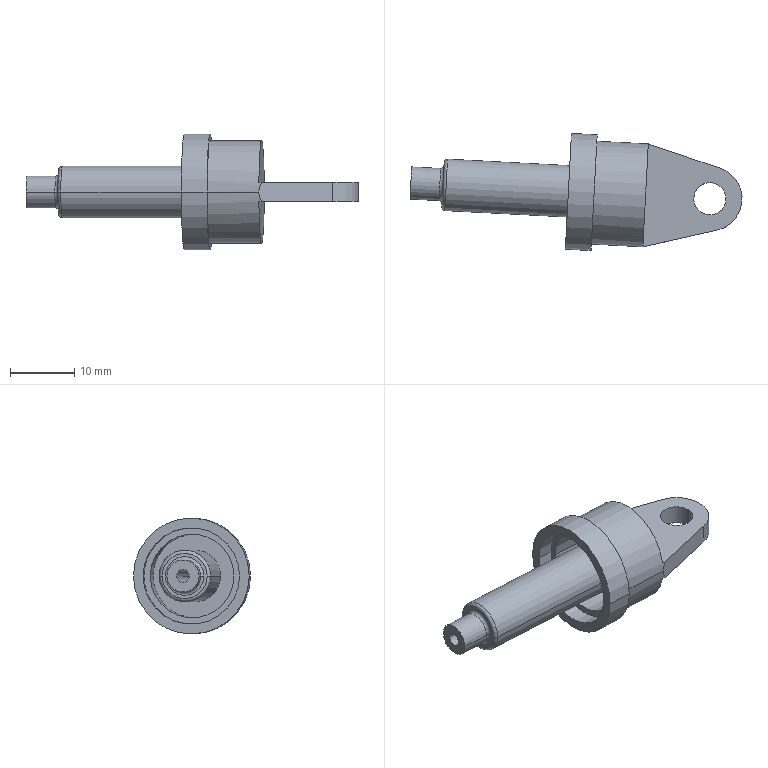Component | SolidWorks | WheelAssembly-1_DamperLowerEnd-1 | 1 solid | 34 faces | box 51.57 x 18.19 x 18 mm | volume 3074 mm3 | cylinder 17 | plane 13 | torus 4 | commonest cylinder face diameters 5 x4 2 x2 13 x2 15 x2 16 x2 18 x2 8 x2 10 x1
build123d program:
from build123d import *

# Parameters (mm, degrees)
SKETCH1_R           = 9
BOSS_EXTRUDE1_DEPTH = 12
CUT_EXTRUDE1_START  = -8
SKETCH2_R           = 9
SKETCH2_R_2         = 8
CUT_EXTRUDE1_DEPTH  = 8
SHELL1_T            = -1.5
SKETCH3_R           = 2.5
BOSS_EXTRUDE2_DEPTH = 1.5
SKETCH4_R           = 9.818
SKETCH4_R_2         = 8
CUT_EXTRUDE2_DEPTH  = 3
SKETCH5_R           = 4
SKETCH5_R_2         = 1
BOSS_EXTRUDE3_DEPTH = 35
CUT_EXTRUDE3_START  = -5
SKETCH6_R           = 4
SKETCH6_R_2         = 2.5
CUT_EXTRUDE3_DEPTH  = 5
FILLET1_R           = 0.5


with BuildPart() as part:
    # Sketch1 → Boss-Extrude1 (new body)
    with BuildSketch(Plane.XY):
        Circle(SKETCH1_R)
    extrude(amount=BOSS_EXTRUDE1_DEPTH)

    # Sketch2 → Cut-Extrude1 (cut)
    with BuildSketch(Plane.XY.offset(12).offset(CUT_EXTRUDE1_START)):
        Circle(SKETCH2_R)
        Circle(SKETCH2_R_2, mode=Mode.SUBTRACT)
    extrude(amount=CUT_EXTRUDE1_DEPTH, mode=Mode.SUBTRACT)

    # Shell1
    shell1_openings = [part.faces().sort_by_distance(p)[0] for p in [
        (0, 0, 0),
    ]]
    offset(amount=SHELL1_T, openings=shell1_openings, kind=Kind.INTERSECTION)

    # Sketch3 → Boss-Extrude2 (add, symmetric)
    with BuildSketch(Plane(origin=(0, 0, 0), x_dir=(1, 0, 0), z_dir=(0, 1, 0))):
        with BuildLine():
            Line((-8, -12), (-4.814, -23.351))
            ThreePointArc((-4.814, -23.351), (0, -27), (4.814, -23.351))
            Line((4.814, -23.351), (8, -12))
            Line((8, -12), (-8, -12))
        make_face()
        with Locations(Location((0, -22, 0), (0, 0, 270))):
            Circle(SKETCH3_R, mode=Mode.SUBTRACT)
    extrude(amount=BOSS_EXTRUDE2_DEPTH, both=True)

    # Sketch4 → Cut-Extrude2 (cut)
    with BuildSketch(Plane.XY.offset(12)):
        Circle(SKETCH4_R)
        Circle(SKETCH4_R_2, mode=Mode.SUBTRACT)
    extrude(amount=CUT_EXTRUDE2_DEPTH, mode=Mode.SUBTRACT)

    # Sketch5 → Boss-Extrude3 (add)
    with BuildSketch(Plane(origin=(0, 0, 10.5), x_dir=(-1, 0, 0), z_dir=(0, 0, -1))):
        with Locations(Location((0, 0, 0), (0, 0, 180))):
            Circle(SKETCH5_R)
        Circle(SKETCH5_R_2, mode=Mode.SUBTRACT)
    extrude(amount=BOSS_EXTRUDE3_DEPTH)

    # Sketch6 → Cut-Extrude3 (cut)
    with BuildSketch(Plane(origin=(0, 0, -24.5), x_dir=(-1, 0, 0), z_dir=(0, 0, -1)).offset(CUT_EXTRUDE3_START)):
        with Locations(Location((0, 0, 0), (0, 0, 180))):
            Circle(SKETCH6_R)
        Circle(SKETCH6_R_2, mode=Mode.SUBTRACT)
    extrude(amount=CUT_EXTRUDE3_DEPTH, mode=Mode.SUBTRACT)

    # Fillet1
    fillet1_edges = [part.edges().sort_by_distance(p)[0] for p in [
        (-4, 0, -19.5),
        (2.5, 0, -19.5),
    ]]
    fillet(fillet1_edges, radius=FILLET1_R)


solid = part.part

# Placed as in the assembly
solid = solid.moved(Location((-279.888, -132.387, -560.47), (90, 86.976, 0)))
STEP:
#1=COLOUR_RGB('',0.7922,0.8196,0.9333);
#2=FILL_AREA_STYLE_COLOUR('',#1);
#3=FILL_AREA_STYLE('',(#2));
#4=SURFACE_STYLE_FILL_AREA(#3);
#5=SURFACE_SIDE_STYLE('',(#4));
#6=SURFACE_STYLE_USAGE(.BOTH.,#5);
#7=PRESENTATION_STYLE_ASSIGNMENT((#6));
#8=CARTESIAN_POINT('',(-11.775,-5.33,-22.066));
#9=VERTEX_POINT('',#8);
#10=CARTESIAN_POINT('',(-11.758,-5.015,-22.066));
#11=VERTEX_POINT('',#10);
#12=CARTESIAN_POINT('',(-11.766,-5.173,-22.066));
#13=DIRECTION('',(0.9986,-0.05275,-0.));
#14=DIRECTION('',(0.05275,0.9986,0.));
#15=AXIS2_PLACEMENT_3D('',#12,#13,#14);
#16=CIRCLE('',#15,0.1575);
#17=EDGE_CURVE('',#9,#11,#16,.T.);
#18=ORIENTED_EDGE('',*,*,#17,.F.);
#19=CARTESIAN_POINT('',(-11.793,-5.309,-22.066));
#20=VERTEX_POINT('',#19);
#21=CARTESIAN_POINT('',(-11.773,-5.31,-22.066));
#22=DIRECTION('',(-0.,-0.,-1.));
#23=DIRECTION('',(0.,1.,0.));
#24=AXIS2_PLACEMENT_3D('',#21,#22,#23);
#25=CIRCLE('',#24,0.01969);
#26=EDGE_CURVE('',#9,#20,#25,.T.);
#27=ORIENTED_EDGE('',*,*,#26,.T.);
#28=CARTESIAN_POINT('',(-11.779,-5.034,-22.066));
#29=VERTEX_POINT('',#28);
#30=CARTESIAN_POINT('',(-11.786,-5.172,-22.066));
#31=DIRECTION('',(-0.9986,0.05275,0.));
#32=DIRECTION('',(0.05275,0.9986,0.));
#33=AXIS2_PLACEMENT_3D('',#30,#31,#32);
#34=CIRCLE('',#33,0.1378);
#35=EDGE_CURVE('',#29,#20,#34,.T.);
#36=ORIENTED_EDGE('',*,*,#35,.F.);
#37=CARTESIAN_POINT('',(-11.759,-5.035,-22.066));
#38=DIRECTION('',(0.,0.,1.));
#39=DIRECTION('',(0.,-1.,0.));
#40=AXIS2_PLACEMENT_3D('',#37,#38,#39);
#41=CIRCLE('',#40,0.01969);
#42=EDGE_CURVE('',#11,#29,#41,.T.);
#43=ORIENTED_EDGE('',*,*,#42,.F.);
#44=EDGE_LOOP('',(#18,#27,#36,#43));
#45=FACE_OUTER_BOUND('',#44,.T.);
#46=CARTESIAN_POINT('',(-11.766,-5.173,-22.066));
#47=DIRECTION('',(-0.9986,0.05275,0.));
#48=DIRECTION('',(0.05275,0.9986,-0.));
#49=AXIS2_PLACEMENT_3D('',#46,#47,#48);
#50=TOROIDAL_SURFACE('',#49,0.1378,0.01969);
#51=ADVANCED_FACE('',(#45),#50,.T.);
#52=CARTESIAN_POINT('',(-11.811,-5.269,-22.066));
#53=VERTEX_POINT('',#52);
#54=CARTESIAN_POINT('',(-11.8,-5.072,-22.066));
#55=VERTEX_POINT('',#54);
#56=CARTESIAN_POINT('',(-11.806,-5.171,-22.066));
#57=DIRECTION('',(-0.9986,0.05275,0.));
#58=DIRECTION('',(0.05275,0.9986,0.));
#59=AXIS2_PLACEMENT_3D('',#56,#57,#58);
#60=CIRCLE('',#59,0.09843);
#61=EDGE_CURVE('',#53,#55,#60,.T.);
#62=ORIENTED_EDGE('',*,*,#61,.F.);
#63=CARTESIAN_POINT('',(-11.792,-5.29,-22.066));
#64=VERTEX_POINT('',#63);
#65=CARTESIAN_POINT('',(-11.812,-5.288,-22.066));
#66=DIRECTION('',(-0.,-0.,-1.));
#67=DIRECTION('',(0.,1.,0.));
#68=AXIS2_PLACEMENT_3D('',#65,#66,#67);
#69=CIRCLE('',#68,0.01969);
#70=EDGE_CURVE('',#53,#64,#69,.T.);
#71=ORIENTED_EDGE('',*,*,#70,.T.);
#72=CARTESIAN_POINT('',(-11.78,-5.054,-22.066));
#73=VERTEX_POINT('',#72);
#74=CARTESIAN_POINT('',(-11.786,-5.172,-22.066));
#75=DIRECTION('',(0.9986,-0.05275,-0.));
#76=DIRECTION('',(0.05275,0.9986,0.));
#77=AXIS2_PLACEMENT_3D('',#74,#75,#76);
#78=CIRCLE('',#77,0.1181);
#79=EDGE_CURVE('',#73,#64,#78,.T.);
#80=ORIENTED_EDGE('',*,*,#79,.F.);
#81=CARTESIAN_POINT('',(-11.799,-5.053,-22.066));
#82=DIRECTION('',(0.,0.,1.));
#83=DIRECTION('',(0.,-1.,0.));
#84=AXIS2_PLACEMENT_3D('',#81,#82,#83);
#85=CIRCLE('',#84,0.01969);
#86=EDGE_CURVE('',#55,#73,#85,.T.);
#87=ORIENTED_EDGE('',*,*,#86,.F.);
#88=EDGE_LOOP('',(#62,#71,#80,#87));
#89=FACE_OUTER_BOUND('',#88,.T.);
#90=CARTESIAN_POINT('',(-11.806,-5.171,-22.066));
#91=DIRECTION('',(-0.9986,0.05275,0.));
#92=DIRECTION('',(0.05275,0.9986,-0.));
#93=AXIS2_PLACEMENT_3D('',#90,#91,#92);
#94=TOROIDAL_SURFACE('',#93,0.1181,0.01969);
#95=ADVANCED_FACE('',(#89),#94,.F.);
#96=CARTESIAN_POINT('',(-11.985,-5.201,-22.066));
#97=VERTEX_POINT('',#96);
#98=CARTESIAN_POINT('',(-11.98,-5.122,-22.066));
#99=VERTEX_POINT('',#98);
#100=CARTESIAN_POINT('',(-11.982,-5.161,-22.066));
#101=DIRECTION('',(-0.9986,0.05275,0.));
#102=DIRECTION('',(0.05275,0.9986,0.));
#103=AXIS2_PLACEMENT_3D('',#100,#101,#102);
#104=CIRCLE('',#103,0.03937);
#105=EDGE_CURVE('',#97,#99,#104,.T.);
#106=ORIENTED_EDGE('',*,*,#105,.T.);
#107=CARTESIAN_POINT('',(-10.604,-5.195,-22.066));
#108=VERTEX_POINT('',#107);
#109=CARTESIAN_POINT('',(-11.98,-5.122,-22.066));
#110=DIRECTION('',(0.9986,-0.05275,-0.));
#111=VECTOR('',#110,39.37);
#112=LINE('',#109,#111);
#113=EDGE_CURVE('',#99,#108,#112,.T.);
#114=ORIENTED_EDGE('',*,*,#113,.T.);
#115=CARTESIAN_POINT('',(-10.608,-5.273,-22.066));
#116=VERTEX_POINT('',#115);
#117=CARTESIAN_POINT('',(-10.606,-5.234,-22.066));
#118=DIRECTION('',(-0.9986,0.05275,0.));
#119=DIRECTION('',(0.05275,0.9986,0.));
#120=AXIS2_PLACEMENT_3D('',#117,#118,#119);
#121=CIRCLE('',#120,0.03937);
#122=EDGE_CURVE('',#116,#108,#121,.T.);
#123=ORIENTED_EDGE('',*,*,#122,.F.);
#124=CARTESIAN_POINT('',(-11.985,-5.201,-22.066));
#125=DIRECTION('',(0.9986,-0.05275,-0.));
#126=VECTOR('',#125,39.37);
#127=LINE('',#124,#126);
#128=EDGE_CURVE('',#97,#116,#127,.T.);
#129=ORIENTED_EDGE('',*,*,#128,.F.);
#130=EDGE_LOOP('',(#106,#114,#123,#129));
#131=FACE_OUTER_BOUND('',#130,.T.);
#132=CARTESIAN_POINT('',(-11.982,-5.161,-22.066));
#133=DIRECTION('',(0.9986,-0.05275,-0.));
#134=DIRECTION('',(-0.05275,-0.9986,0.));
#135=AXIS2_PLACEMENT_3D('',#132,#133,#134);
#136=CYLINDRICAL_SURFACE('',#135,0.03937);
#137=ADVANCED_FACE('',(#131),#136,.F.);
#138=CARTESIAN_POINT('',(-11.806,-5.171,-22.066));
#139=DIRECTION('',(-0.9986,0.05275,0.));
#140=DIRECTION('',(0.05275,0.9986,0.));
#141=AXIS2_PLACEMENT_3D('',#138,#139,#140);
#142=CIRCLE('',#141,0.09843);
#143=EDGE_CURVE('',#55,#53,#142,.T.);
#144=ORIENTED_EDGE('',*,*,#143,.T.);
#145=CARTESIAN_POINT('',(-11.988,-5.259,-22.066));
#146=VERTEX_POINT('',#145);
#147=CARTESIAN_POINT('',(-11.791,-5.27,-22.066));
#148=DIRECTION('',(-0.9986,0.05275,0.));
#149=VECTOR('',#148,39.37);
#150=LINE('',#147,#149);
#151=EDGE_CURVE('',#53,#146,#150,.T.);
#152=ORIENTED_EDGE('',*,*,#151,.T.);
#153=CARTESIAN_POINT('',(-11.977,-5.063,-22.066));
#154=VERTEX_POINT('',#153);
#155=CARTESIAN_POINT('',(-11.982,-5.161,-22.066));
#156=DIRECTION('',(-0.9986,0.05275,0.));
#157=DIRECTION('',(0.05275,0.9986,0.));
#158=AXIS2_PLACEMENT_3D('',#155,#156,#157);
#159=CIRCLE('',#158,0.09843);
#160=EDGE_CURVE('',#154,#146,#159,.T.);
#161=ORIENTED_EDGE('',*,*,#160,.F.);
#162=CARTESIAN_POINT('',(-11.781,-5.073,-22.066));
#163=DIRECTION('',(-0.9986,0.05275,0.));
#164=VECTOR('',#163,39.37);
#165=LINE('',#162,#164);
#166=EDGE_CURVE('',#55,#154,#165,.T.);
#167=ORIENTED_EDGE('',*,*,#166,.F.);
#168=EDGE_LOOP('',(#144,#152,#161,#167));
#169=FACE_OUTER_BOUND('',#168,.T.);
#170=CARTESIAN_POINT('',(-11.786,-5.172,-22.066));
#171=DIRECTION('',(-0.9986,0.05275,0.));
#172=DIRECTION('',(0.05275,0.9986,0.));
#173=AXIS2_PLACEMENT_3D('',#170,#171,#172);
#174=CYLINDRICAL_SURFACE('',#173,0.09843);
#175=ADVANCED_FACE('',(#169),#174,.T.);
#176=CARTESIAN_POINT('',(-10.253,-5.253,-22.125));
#177=VERTEX_POINT('',#176);
#178=CARTESIAN_POINT('',(-10.056,-5.263,-22.125));
#179=VERTEX_POINT('',#178);
#180=CARTESIAN_POINT('',(-10.154,-5.258,-22.125));
#181=DIRECTION('',(-0.,-0.,-1.));
#182=DIRECTION('',(0.9986,-0.05275,0.));
#183=AXIS2_PLACEMENT_3D('',#180,#181,#182);
#184=CIRCLE('',#183,0.09843);
#185=EDGE_CURVE('',#177,#179,#184,.T.);
#186=ORIENTED_EDGE('',*,*,#185,.T.);
#187=CARTESIAN_POINT('',(-10.056,-5.263,-22.007));
#188=VERTEX_POINT('',#187);
#189=CARTESIAN_POINT('',(-10.056,-5.263,-22.125));
#190=DIRECTION('',(0.,0.,1.));
#191=VECTOR('',#190,39.37);
#192=LINE('',#189,#191);
#193=EDGE_CURVE('',#179,#188,#192,.T.);
#194=ORIENTED_EDGE('',*,*,#193,.T.);
#195=CARTESIAN_POINT('',(-10.253,-5.253,-22.007));
#196=VERTEX_POINT('',#195);
#197=CARTESIAN_POINT('',(-10.154,-5.258,-22.007));
#198=DIRECTION('',(-0.,-0.,-1.));
#199=DIRECTION('',(0.9986,-0.05275,0.));
#200=AXIS2_PLACEMENT_3D('',#197,#198,#199);
#201=CIRCLE('',#200,0.09843);
#202=EDGE_CURVE('',#196,#188,#201,.T.);
#203=ORIENTED_EDGE('',*,*,#202,.F.);
#204=CARTESIAN_POINT('',(-10.253,-5.253,-22.125));
#205=DIRECTION('',(0.,0.,1.));
#206=VECTOR('',#205,39.37);
#207=LINE('',#204,#206);
#208=EDGE_CURVE('',#177,#196,#207,.T.);
#209=ORIENTED_EDGE('',*,*,#208,.F.);
#210=EDGE_LOOP('',(#186,#194,#203,#209));
#211=FACE_OUTER_BOUND('',#210,.T.);
#212=CARTESIAN_POINT('',(-10.154,-5.258,-22.125));
#213=DIRECTION('',(0.,0.,1.));
#214=DIRECTION('',(-0.9986,0.05275,0.));
#215=AXIS2_PLACEMENT_3D('',#212,#213,#214);
#216=CYLINDRICAL_SURFACE('',#215,0.09843);
#217=ADVANCED_FACE('',(#211),#216,.F.);
#218=CARTESIAN_POINT('',(-10.907,-4.962,-22.066));
#219=VERTEX_POINT('',#218);
#220=CARTESIAN_POINT('',(-10.934,-5.473,-22.066));
#221=VERTEX_POINT('',#220);
#222=CARTESIAN_POINT('',(-10.921,-5.217,-22.066));
#223=DIRECTION('',(0.9986,-0.05275,-0.));
#224=DIRECTION('',(-0.05275,-0.9986,0.));
#225=AXIS2_PLACEMENT_3D('',#222,#223,#224);
#226=CIRCLE('',#225,0.2559);
#227=EDGE_CURVE('',#219,#221,#226,.T.);
#228=ORIENTED_EDGE('',*,*,#227,.F.);
#229=CARTESIAN_POINT('',(-10.593,-4.978,-22.066));
#230=VERTEX_POINT('',#229);
#231=CARTESIAN_POINT('',(-10.848,-4.965,-22.066));
#232=DIRECTION('',(0.9986,-0.05275,-0.));
#233=VECTOR('',#232,39.37);
#234=LINE('',#231,#233);
#235=EDGE_CURVE('',#219,#230,#234,.T.);
#236=ORIENTED_EDGE('',*,*,#235,.T.);
#237=CARTESIAN_POINT('',(-10.62,-5.489,-22.066));
#238=VERTEX_POINT('',#237);
#239=CARTESIAN_POINT('',(-10.606,-5.234,-22.066));
#240=DIRECTION('',(0.9986,-0.05275,-0.));
#241=DIRECTION('',(-0.05275,-0.9986,0.));
#242=AXIS2_PLACEMENT_3D('',#239,#240,#241);
#243=CIRCLE('',#242,0.2559);
#244=EDGE_CURVE('',#230,#238,#243,.T.);
#245=ORIENTED_EDGE('',*,*,#244,.T.);
#246=CARTESIAN_POINT('',(-10.875,-5.476,-22.066));
#247=DIRECTION('',(0.9986,-0.05275,-0.));
#248=VECTOR('',#247,39.37);
#249=LINE('',#246,#248);
#250=EDGE_CURVE('',#221,#238,#249,.T.);
#251=ORIENTED_EDGE('',*,*,#250,.F.);
#252=EDGE_LOOP('',(#228,#236,#245,#251));
#253=FACE_OUTER_BOUND('',#252,.T.);
#254=CARTESIAN_POINT('',(-10.862,-5.22,-22.066));
#255=DIRECTION('',(0.9986,-0.05275,-0.));
#256=DIRECTION('',(-0.05275,-0.9986,0.));
#257=AXIS2_PLACEMENT_3D('',#254,#255,#256);
#258=CYLINDRICAL_SURFACE('',#257,0.2559);
#259=ADVANCED_FACE('',(#253),#258,.F.);
#260=CARTESIAN_POINT('',(-10.905,-4.922,-22.066));
#261=VERTEX_POINT('',#260);
#262=CARTESIAN_POINT('',(-10.937,-5.512,-22.066));
#263=VERTEX_POINT('',#262);
#264=CARTESIAN_POINT('',(-10.921,-5.217,-22.066));
#265=DIRECTION('',(0.9986,-0.05275,-0.));
#266=DIRECTION('',(-0.05275,-0.9986,0.));
#267=AXIS2_PLACEMENT_3D('',#264,#265,#266);
#268=CIRCLE('',#267,0.2953);
#269=EDGE_CURVE('',#261,#263,#268,.T.);
#270=ORIENTED_EDGE('',*,*,#269,.T.);
#271=CARTESIAN_POINT('',(-11.035,-5.507,-22.066));
#272=VERTEX_POINT('',#271);
#273=CARTESIAN_POINT('',(-10.563,-5.532,-22.066));
#274=DIRECTION('',(-0.9986,0.05275,0.));
#275=VECTOR('',#274,39.37);
#276=LINE('',#273,#275);
#277=EDGE_CURVE('',#263,#272,#276,.T.);
#278=ORIENTED_EDGE('',*,*,#277,.T.);
#279=CARTESIAN_POINT('',(-11.004,-4.917,-22.066));
#280=VERTEX_POINT('',#279);
#281=CARTESIAN_POINT('',(-11.019,-5.212,-22.066));
#282=DIRECTION('',(0.9986,-0.05275,-0.));
#283=DIRECTION('',(-0.05275,-0.9986,0.));
#284=AXIS2_PLACEMENT_3D('',#281,#282,#283);
#285=CIRCLE('',#284,0.2953);
#286=EDGE_CURVE('',#280,#272,#285,.T.);
#287=ORIENTED_EDGE('',*,*,#286,.F.);
#288=CARTESIAN_POINT('',(-10.532,-4.942,-22.066));
#289=DIRECTION('',(-0.9986,0.05275,0.));
#290=VECTOR('',#289,39.37);
#291=LINE('',#288,#290);
#292=EDGE_CURVE('',#261,#280,#291,.T.);
#293=ORIENTED_EDGE('',*,*,#292,.F.);
#294=EDGE_LOOP('',(#270,#278,#287,#293));
#295=FACE_OUTER_BOUND('',#294,.T.);
#296=CARTESIAN_POINT('',(-10.547,-5.237,-22.066));
#297=DIRECTION('',(-0.9986,0.05275,0.));
#298=DIRECTION('',(0.05275,0.9986,0.));
#299=AXIS2_PLACEMENT_3D('',#296,#297,#298);
#300=CYLINDRICAL_SURFACE('',#299,0.2953);
#301=ADVANCED_FACE('',(#295),#300,.F.);
#302=CARTESIAN_POINT('',(-10.879,-5.535,-22.066));
#303=VERTEX_POINT('',#302);
#304=CARTESIAN_POINT('',(-10.845,-4.906,-22.066));
#305=VERTEX_POINT('',#304);
#306=CARTESIAN_POINT('',(-10.862,-5.22,-22.066));
#307=DIRECTION('',(0.9986,-0.05275,-0.));
#308=DIRECTION('',(-0.05275,-0.9986,0.));
#309=AXIS2_PLACEMENT_3D('',#306,#307,#308);
#310=CIRCLE('',#309,0.315);
#311=EDGE_CURVE('',#303,#305,#310,.T.);
#312=ORIENTED_EDGE('',*,*,#311,.T.);
#313=CARTESIAN_POINT('',(-10.531,-4.922,-22.066));
#314=VERTEX_POINT('',#313);
#315=CARTESIAN_POINT('',(-10.845,-4.906,-22.066));
#316=DIRECTION('',(0.9986,-0.05275,-0.));
#317=VECTOR('',#316,39.37);
#318=LINE('',#315,#317);
#319=EDGE_CURVE('',#305,#314,#318,.T.);
#320=ORIENTED_EDGE('',*,*,#319,.T.);
#321=CARTESIAN_POINT('',(-10.511,-4.929,-22.125));
#322=VERTEX_POINT('',#321);
#323=CARTESIAN_POINT('',(-10.511,-4.929,-22.125));
#324=CARTESIAN_POINT('',(-10.524,-4.925,-22.105));
#325=CARTESIAN_POINT('',(-10.531,-4.922,-22.086));
#326=CARTESIAN_POINT('',(-10.531,-4.922,-22.066));
#327=(BOUNDED_CURVE()B_SPLINE_CURVE(3,(#323,#324,#325,#326),.UNSPECIFIED.,.F.,.F.)B_SPLINE_CURVE_WITH_KNOTS((4,4),(6.095,6.283),.UNSPECIFIED.)CURVE()GEOMETRIC_REPRESENTATION_ITEM()RATIONAL_B_SPLINE_CURVE((1.,0.997,0.997,1.))REPRESENTATION_ITEM(''));
#328=EDGE_CURVE('',#322,#314,#327,.T.);
#329=ORIENTED_EDGE('',*,*,#328,.F.);
#330=CARTESIAN_POINT('',(-10.531,-4.928,-22.125));
#331=VERTEX_POINT('',#330);
#332=CARTESIAN_POINT('',(-10.413,-4.934,-22.125));
#333=DIRECTION('',(-0.9986,0.05275,0.));
#334=VECTOR('',#333,39.37);
#335=LINE('',#332,#334);
#336=EDGE_CURVE('',#322,#331,#335,.T.);
#337=ORIENTED_EDGE('',*,*,#336,.T.);
#338=CARTESIAN_POINT('',(-10.564,-5.546,-22.125));
#339=VERTEX_POINT('',#338);
#340=CARTESIAN_POINT('',(-10.547,-5.237,-22.066));
#341=DIRECTION('',(0.9986,-0.05275,-0.));
#342=DIRECTION('',(-0.05275,-0.9986,0.));
#343=AXIS2_PLACEMENT_3D('',#340,#341,#342);
#344=CIRCLE('',#343,0.315);
#345=EDGE_CURVE('',#339,#331,#344,.T.);
#346=ORIENTED_EDGE('',*,*,#345,.F.);
#347=CARTESIAN_POINT('',(-10.544,-5.547,-22.125));
#348=VERTEX_POINT('',#347);
#349=CARTESIAN_POINT('',(-10.446,-5.552,-22.125));
#350=DIRECTION('',(0.9986,-0.05275,-0.));
#351=VECTOR('',#350,39.37);
#352=LINE('',#349,#351);
#353=EDGE_CURVE('',#339,#348,#352,.T.);
#354=ORIENTED_EDGE('',*,*,#353,.T.);
#355=CARTESIAN_POINT('',(-10.564,-5.552,-22.066));
#356=VERTEX_POINT('',#355);
#357=CARTESIAN_POINT('',(-10.564,-5.552,-22.066));
#358=CARTESIAN_POINT('',(-10.564,-5.552,-22.086));
#359=CARTESIAN_POINT('',(-10.557,-5.55,-22.105));
#360=CARTESIAN_POINT('',(-10.544,-5.547,-22.125));
#361=(BOUNDED_CURVE()B_SPLINE_CURVE(3,(#357,#358,#359,#360),.UNSPECIFIED.,.F.,.F.)B_SPLINE_CURVE_WITH_KNOTS((4,4),(0.,0.1886),.UNSPECIFIED.)CURVE()GEOMETRIC_REPRESENTATION_ITEM()RATIONAL_B_SPLINE_CURVE((1.,0.997,0.997,1.))REPRESENTATION_ITEM(''));
#362=EDGE_CURVE('',#356,#348,#361,.T.);
#363=ORIENTED_EDGE('',*,*,#362,.F.);
#364=CARTESIAN_POINT('',(-10.879,-5.535,-22.066));
#365=DIRECTION('',(0.9986,-0.05275,-0.));
#366=VECTOR('',#365,39.37);
#367=LINE('',#364,#366);
#368=EDGE_CURVE('',#303,#356,#367,.T.);
#369=ORIENTED_EDGE('',*,*,#368,.F.);
#370=EDGE_LOOP('',(#312,#320,#329,#337,#346,#354,#363,#369));
#371=FACE_OUTER_BOUND('',#370,.T.);
#372=CARTESIAN_POINT('',(-10.862,-5.22,-22.066));
#373=DIRECTION('',(0.9986,-0.05275,-0.));
#374=DIRECTION('',(-0.05275,-0.9986,0.));
#375=AXIS2_PLACEMENT_3D('',#372,#373,#374);
#376=CYLINDRICAL_SURFACE('',#375,0.315);
#377=ADVANCED_FACE('',(#371),#376,.T.);
#378=CARTESIAN_POINT('',(-10.881,-5.574,-22.066));
#379=VERTEX_POINT('',#378);
#380=CARTESIAN_POINT('',(-10.843,-4.867,-22.066));
#381=VERTEX_POINT('',#380);
#382=CARTESIAN_POINT('',(-10.862,-5.22,-22.066));
#383=DIRECTION('',(0.9986,-0.05275,-0.));
#384=DIRECTION('',(-0.05275,-0.9986,0.));
#385=AXIS2_PLACEMENT_3D('',#382,#383,#384);
#386=CIRCLE('',#385,0.3543);
#387=EDGE_CURVE('',#379,#381,#386,.T.);
#388=ORIENTED_EDGE('',*,*,#387,.F.);
#389=CARTESIAN_POINT('',(-11.038,-5.566,-22.066));
#390=VERTEX_POINT('',#389);
#391=CARTESIAN_POINT('',(-10.566,-5.591,-22.066));
#392=DIRECTION('',(-0.9986,0.05275,0.));
#393=VECTOR('',#392,39.37);
#394=LINE('',#391,#393);
#395=EDGE_CURVE('',#379,#390,#394,.T.);
#396=ORIENTED_EDGE('',*,*,#395,.T.);
#397=CARTESIAN_POINT('',(-11.001,-4.858,-22.066));
#398=VERTEX_POINT('',#397);
#399=CARTESIAN_POINT('',(-11.019,-5.212,-22.066));
#400=DIRECTION('',(0.9986,-0.05275,-0.));
#401=DIRECTION('',(-0.05275,-0.9986,0.));
#402=AXIS2_PLACEMENT_3D('',#399,#400,#401);
#403=CIRCLE('',#402,0.3543);
#404=EDGE_CURVE('',#390,#398,#403,.T.);
#405=ORIENTED_EDGE('',*,*,#404,.T.);
#406=CARTESIAN_POINT('',(-10.529,-4.883,-22.066));
#407=DIRECTION('',(-0.9986,0.05275,0.));
#408=VECTOR('',#407,39.37);
#409=LINE('',#406,#408);
#410=EDGE_CURVE('',#381,#398,#409,.T.);
#411=ORIENTED_EDGE('',*,*,#410,.F.);
#412=EDGE_LOOP('',(#388,#396,#405,#411));
#413=FACE_OUTER_BOUND('',#412,.T.);
#414=CARTESIAN_POINT('',(-10.547,-5.237,-22.066));
#415=DIRECTION('',(-0.9986,0.05275,0.));
#416=DIRECTION('',(0.05275,0.9986,0.));
#417=AXIS2_PLACEMENT_3D('',#414,#415,#416);
#418=CYLINDRICAL_SURFACE('',#417,0.3543);
#419=ADVANCED_FACE('',(#413),#418,.T.);
#420=ORIENTED_EDGE('',*,*,#17,.T.);
#421=CARTESIAN_POINT('',(-10.598,-5.077,-22.066));
#422=VERTEX_POINT('',#421);
#423=CARTESIAN_POINT('',(-11.974,-5.004,-22.066));
#424=DIRECTION('',(0.9986,-0.05275,-0.));
#425=VECTOR('',#424,39.37);
#426=LINE('',#423,#425);
#427=EDGE_CURVE('',#11,#422,#426,.T.);
#428=ORIENTED_EDGE('',*,*,#427,.T.);
#429=CARTESIAN_POINT('',(-10.615,-5.391,-22.066));
#430=VERTEX_POINT('',#429);
#431=CARTESIAN_POINT('',(-10.606,-5.234,-22.066));
#432=DIRECTION('',(-0.9986,0.05275,0.));
#433=DIRECTION('',(-0.05275,-0.9986,0.));
#434=AXIS2_PLACEMENT_3D('',#431,#432,#433);
#435=CIRCLE('',#434,0.1575);
#436=EDGE_CURVE('',#422,#430,#435,.T.);
#437=ORIENTED_EDGE('',*,*,#436,.T.);
#438=CARTESIAN_POINT('',(-11.991,-5.318,-22.066));
#439=DIRECTION('',(0.9986,-0.05275,-0.));
#440=VECTOR('',#439,39.37);
#441=LINE('',#438,#440);
#442=EDGE_CURVE('',#9,#430,#441,.T.);
#443=ORIENTED_EDGE('',*,*,#442,.F.);
#444=EDGE_LOOP('',(#420,#428,#437,#443));
#445=FACE_OUTER_BOUND('',#444,.T.);
#446=CARTESIAN_POINT('',(-11.982,-5.161,-22.066));
#447=DIRECTION('',(0.9986,-0.05275,-0.));
#448=DIRECTION('',(-0.05275,-0.9986,0.));
#449=AXIS2_PLACEMENT_3D('',#446,#447,#448);
#450=CYLINDRICAL_SURFACE('',#449,0.1575);
#451=ADVANCED_FACE('',(#445),#450,.T.);
#452=ORIENTED_EDGE('',*,*,#427,.F.);
#453=CARTESIAN_POINT('',(-11.766,-5.173,-22.066));
#454=DIRECTION('',(0.9986,-0.05275,-0.));
#455=DIRECTION('',(0.05275,0.9986,0.));
#456=AXIS2_PLACEMENT_3D('',#453,#454,#455);
#457=CIRCLE('',#456,0.1575);
#458=EDGE_CURVE('',#11,#9,#457,.T.);
#459=ORIENTED_EDGE('',*,*,#458,.T.);
#460=ORIENTED_EDGE('',*,*,#442,.T.);
#461=CARTESIAN_POINT('',(-10.606,-5.234,-22.066));
#462=DIRECTION('',(-0.9986,0.05275,0.));
#463=DIRECTION('',(-0.05275,-0.9986,0.));
#464=AXIS2_PLACEMENT_3D('',#461,#462,#463);
#465=CIRCLE('',#464,0.1575);
#466=EDGE_CURVE('',#430,#422,#465,.T.);
#467=ORIENTED_EDGE('',*,*,#466,.T.);
#468=EDGE_LOOP('',(#452,#459,#460,#467));
#469=FACE_OUTER_BOUND('',#468,.T.);
#470=CARTESIAN_POINT('',(-11.982,-5.161,-22.066));
#471=DIRECTION('',(0.9986,-0.05275,-0.));
#472=DIRECTION('',(-0.05275,-0.9986,0.));
#473=AXIS2_PLACEMENT_3D('',#470,#471,#472);
#474=CYLINDRICAL_SURFACE('',#473,0.1575);
#475=ADVANCED_FACE('',(#469),#474,.T.);
#476=CARTESIAN_POINT('',(-10.091,-5.071,-22.125));
#477=VERTEX_POINT('',#476);
#478=CARTESIAN_POINT('',(-10.531,-4.922,-22.125));
#479=DIRECTION('',(0.9472,-0.3206,0.));
#480=VECTOR('',#479,39.37);
#481=LINE('',#478,#480);
#482=EDGE_CURVE('',#322,#477,#481,.T.);
#483=ORIENTED_EDGE('',*,*,#482,.F.);
#484=ORIENTED_EDGE('',*,*,#328,.T.);
#485=CARTESIAN_POINT('',(-10.511,-4.929,-22.007));
#486=VERTEX_POINT('',#485);
#487=CARTESIAN_POINT('',(-10.531,-4.922,-22.066));
#488=CARTESIAN_POINT('',(-10.531,-4.922,-22.046));
#489=CARTESIAN_POINT('',(-10.524,-4.925,-22.026));
#490=CARTESIAN_POINT('',(-10.511,-4.929,-22.007));
#491=(BOUNDED_CURVE()B_SPLINE_CURVE(3,(#487,#488,#489,#490),.UNSPECIFIED.,.F.,.F.)B_SPLINE_CURVE_WITH_KNOTS((4,4),(0.,0.1886),.UNSPECIFIED.)CURVE()GEOMETRIC_REPRESENTATION_ITEM()RATIONAL_B_SPLINE_CURVE((1.,0.997,0.997,1.))REPRESENTATION_ITEM(''));
#492=EDGE_CURVE('',#314,#486,#491,.T.);
#493=ORIENTED_EDGE('',*,*,#492,.T.);
#494=CARTESIAN_POINT('',(-10.091,-5.071,-22.007));
#495=VERTEX_POINT('',#494);
#496=CARTESIAN_POINT('',(-10.531,-4.922,-22.007));
#497=DIRECTION('',(0.9472,-0.3206,0.));
#498=VECTOR('',#497,39.37);
#499=LINE('',#496,#498);
#500=EDGE_CURVE('',#486,#495,#499,.T.);
#501=ORIENTED_EDGE('',*,*,#500,.T.);
#502=CARTESIAN_POINT('',(-10.091,-5.071,-22.125));
#503=DIRECTION('',(0.,0.,1.));
#504=VECTOR('',#503,39.37);
#505=LINE('',#502,#504);
#506=EDGE_CURVE('',#477,#495,#505,.T.);
#507=ORIENTED_EDGE('',*,*,#506,.F.);
#508=EDGE_LOOP('',(#483,#484,#493,#501,#507));
#509=FACE_OUTER_BOUND('',#508,.T.);
#510=CARTESIAN_POINT('',(-10.531,-4.922,-22.125));
#511=DIRECTION('',(-0.3206,-0.9472,0.));
#512=DIRECTION('',(-0.9472,0.3206,-0.));
#513=AXIS2_PLACEMENT_3D('',#510,#511,#512);
#514=PLANE('',#513);
#515=ADVANCED_FACE('',(#509),#514,.F.);
#516=CARTESIAN_POINT('',(-10.544,-5.547,-22.007));
#517=VERTEX_POINT('',#516);
#518=CARTESIAN_POINT('',(-10.544,-5.547,-22.007));
#519=CARTESIAN_POINT('',(-10.557,-5.55,-22.026));
#520=CARTESIAN_POINT('',(-10.564,-5.552,-22.046));
#521=CARTESIAN_POINT('',(-10.564,-5.552,-22.066));
#522=(BOUNDED_CURVE()B_SPLINE_CURVE(3,(#518,#519,#520,#521),.UNSPECIFIED.,.F.,.F.)B_SPLINE_CURVE_WITH_KNOTS((4,4),(6.095,6.283),.UNSPECIFIED.)CURVE()GEOMETRIC_REPRESENTATION_ITEM()RATIONAL_B_SPLINE_CURVE((1.,0.997,0.997,1.))REPRESENTATION_ITEM(''));
#523=EDGE_CURVE('',#517,#356,#522,.T.);
#524=ORIENTED_EDGE('',*,*,#523,.T.);
#525=ORIENTED_EDGE('',*,*,#362,.T.);
#526=CARTESIAN_POINT('',(-10.111,-5.45,-22.125));
#527=VERTEX_POINT('',#526);
#528=CARTESIAN_POINT('',(-10.564,-5.552,-22.125));
#529=DIRECTION('',(-0.9757,-0.2191,0.));
#530=VECTOR('',#529,39.37);
#531=LINE('',#528,#530);
#532=EDGE_CURVE('',#527,#348,#531,.T.);
#533=ORIENTED_EDGE('',*,*,#532,.F.);
#534=CARTESIAN_POINT('',(-10.111,-5.45,-22.007));
#535=VERTEX_POINT('',#534);
#536=CARTESIAN_POINT('',(-10.111,-5.45,-22.125));
#537=DIRECTION('',(0.,0.,1.));
#538=VECTOR('',#537,39.37);
#539=LINE('',#536,#538);
#540=EDGE_CURVE('',#527,#535,#539,.T.);
#541=ORIENTED_EDGE('',*,*,#540,.T.);
#542=CARTESIAN_POINT('',(-10.564,-5.552,-22.007));
#543=DIRECTION('',(-0.9757,-0.2191,0.));
#544=VECTOR('',#543,39.37);
#545=LINE('',#542,#544);
#546=EDGE_CURVE('',#535,#517,#545,.T.);
#547=ORIENTED_EDGE('',*,*,#546,.T.);
#548=EDGE_LOOP('',(#524,#525,#533,#541,#547));
#549=FACE_OUTER_BOUND('',#548,.T.);
#550=CARTESIAN_POINT('',(-10.564,-5.552,-22.125));
#551=DIRECTION('',(-0.2191,0.9757,-0.));
#552=DIRECTION('',(0.9757,0.2191,-0.));
#553=AXIS2_PLACEMENT_3D('',#550,#551,#552);
#554=PLANE('',#553);
#555=ADVANCED_FACE('',(#549),#554,.F.);
#556=CARTESIAN_POINT('',(-10.531,-4.928,-22.007));
#557=VERTEX_POINT('',#556);
#558=CARTESIAN_POINT('',(-10.564,-5.546,-22.007));
#559=VERTEX_POINT('',#558);
#560=CARTESIAN_POINT('',(-10.547,-5.237,-22.066));
#561=DIRECTION('',(0.9986,-0.05275,-0.));
#562=DIRECTION('',(-0.05275,-0.9986,0.));
#563=AXIS2_PLACEMENT_3D('',#560,#561,#562);
#564=CIRCLE('',#563,0.315);
#565=EDGE_CURVE('',#557,#559,#564,.T.);
#566=ORIENTED_EDGE('',*,*,#565,.T.);
#567=CARTESIAN_POINT('',(-10.531,-4.922,-22.007));
#568=DIRECTION('',(0.05275,0.9986,-0.));
#569=VECTOR('',#568,39.37);
#570=LINE('',#567,#569);
#571=EDGE_CURVE('',#559,#557,#570,.T.);
#572=ORIENTED_EDGE('',*,*,#571,.T.);
#573=EDGE_LOOP('',(#566,#572));
#574=FACE_OUTER_BOUND('',#573,.T.);
#575=CARTESIAN_POINT('',(-10.547,-5.237,-22.066));
#576=DIRECTION('',(0.9986,-0.05275,-0.));
#577=DIRECTION('',(-0.05275,-0.9986,0.));
#578=AXIS2_PLACEMENT_3D('',#575,#576,#577);
#579=PLANE('',#578);
#580=ADVANCED_FACE('',(#574),#579,.T.);
#581=ORIENTED_EDGE('',*,*,#395,.F.);
#582=CARTESIAN_POINT('',(-10.862,-5.22,-22.066));
#583=DIRECTION('',(0.9986,-0.05275,-0.));
#584=DIRECTION('',(-0.05275,-0.9986,0.));
#585=AXIS2_PLACEMENT_3D('',#582,#583,#584);
#586=CIRCLE('',#585,0.3543);
#587=EDGE_CURVE('',#381,#379,#586,.T.);
#588=ORIENTED_EDGE('',*,*,#587,.F.);
#589=ORIENTED_EDGE('',*,*,#410,.T.);
#590=CARTESIAN_POINT('',(-11.019,-5.212,-22.066));
#591=DIRECTION('',(0.9986,-0.05275,-0.));
#592=DIRECTION('',(-0.05275,-0.9986,0.));
#593=AXIS2_PLACEMENT_3D('',#590,#591,#592);
#594=CIRCLE('',#593,0.3543);
#595=EDGE_CURVE('',#398,#390,#594,.T.);
#596=ORIENTED_EDGE('',*,*,#595,.T.);
#597=EDGE_LOOP('',(#581,#588,#589,#596));
#598=FACE_OUTER_BOUND('',#597,.T.);
#599=CARTESIAN_POINT('',(-10.547,-5.237,-22.066));
#600=DIRECTION('',(-0.9986,0.05275,0.));
#601=DIRECTION('',(0.05275,0.9986,0.));
#602=AXIS2_PLACEMENT_3D('',#599,#600,#601);
#603=CYLINDRICAL_SURFACE('',#602,0.3543);
#604=ADVANCED_FACE('',(#598),#603,.T.);
#605=ORIENTED_EDGE('',*,*,#286,.T.);
#606=CARTESIAN_POINT('',(-11.019,-5.212,-22.066));
#607=DIRECTION('',(0.9986,-0.05275,-0.));
#608=DIRECTION('',(-0.05275,-0.9986,0.));
#609=AXIS2_PLACEMENT_3D('',#606,#607,#608);
#610=CIRCLE('',#609,0.2953);
#611=EDGE_CURVE('',#272,#280,#610,.T.);
#612=ORIENTED_EDGE('',*,*,#611,.T.);
#613=EDGE_LOOP('',(#605,#612));
#614=FACE_BOUND('',#613,.T.);
#615=ORIENTED_EDGE('',*,*,#595,.F.);
#616=ORIENTED_EDGE('',*,*,#404,.F.);
#617=EDGE_LOOP('',(#615,#616));
#618=FACE_OUTER_BOUND('',#617,.T.);
#619=CARTESIAN_POINT('',(-11.019,-5.212,-22.066));
#620=DIRECTION('',(0.9986,-0.05275,-0.));
#621=DIRECTION('',(-0.05275,-0.9986,0.));
#622=AXIS2_PLACEMENT_3D('',#619,#620,#621);
#623=PLANE('',#622);
#624=ADVANCED_FACE('',(#614,#618),#623,.F.);
#625=ORIENTED_EDGE('',*,*,#311,.F.);
#626=CARTESIAN_POINT('',(-10.862,-5.22,-22.066));
#627=DIRECTION('',(0.9986,-0.05275,-0.));
#628=DIRECTION('',(-0.05275,-0.9986,0.));
#629=AXIS2_PLACEMENT_3D('',#626,#627,#628);
#630=CIRCLE('',#629,0.315);
#631=EDGE_CURVE('',#305,#303,#630,.T.);
#632=ORIENTED_EDGE('',*,*,#631,.F.);
#633=EDGE_LOOP('',(#625,#632));
#634=FACE_BOUND('',#633,.T.);
#635=ORIENTED_EDGE('',*,*,#587,.T.);
#636=ORIENTED_EDGE('',*,*,#387,.T.);
#637=EDGE_LOOP('',(#635,#636));
#638=FACE_OUTER_BOUND('',#637,.T.);
#639=CARTESIAN_POINT('',(-10.862,-5.22,-22.066));
#640=DIRECTION('',(0.9986,-0.05275,-0.));
#641=DIRECTION('',(-0.05275,-0.9986,0.));
#642=AXIS2_PLACEMENT_3D('',#639,#640,#641);
#643=PLANE('',#642);
#644=ADVANCED_FACE('',(#634,#638),#643,.T.);
#645=ORIENTED_EDGE('',*,*,#319,.F.);
#646=ORIENTED_EDGE('',*,*,#631,.T.);
#647=ORIENTED_EDGE('',*,*,#368,.T.);
#648=ORIENTED_EDGE('',*,*,#523,.F.);
#649=CARTESIAN_POINT('',(-10.446,-5.552,-22.007));
#650=DIRECTION('',(0.9986,-0.05275,-0.));
#651=VECTOR('',#650,39.37);
#652=LINE('',#649,#651);
#653=EDGE_CURVE('',#559,#517,#652,.T.);
#654=ORIENTED_EDGE('',*,*,#653,.F.);
#655=ORIENTED_EDGE('',*,*,#565,.F.);
#656=CARTESIAN_POINT('',(-10.413,-4.934,-22.007));
#657=DIRECTION('',(-0.9986,0.05275,0.));
#658=VECTOR('',#657,39.37);
#659=LINE('',#656,#658);
#660=EDGE_CURVE('',#486,#557,#659,.T.);
#661=ORIENTED_EDGE('',*,*,#660,.F.);
#662=ORIENTED_EDGE('',*,*,#492,.F.);
#663=EDGE_LOOP('',(#645,#646,#647,#648,#654,#655,#661,#662));
#664=FACE_OUTER_BOUND('',#663,.T.);
#665=CARTESIAN_POINT('',(-10.862,-5.22,-22.066));
#666=DIRECTION('',(0.9986,-0.05275,-0.));
#667=DIRECTION('',(-0.05275,-0.9986,0.));
#668=AXIS2_PLACEMENT_3D('',#665,#666,#667);
#669=CYLINDRICAL_SURFACE('',#668,0.315);
#670=ADVANCED_FACE('',(#664),#669,.T.);
#671=CARTESIAN_POINT('',(-10.531,-4.922,-22.125));
#672=DIRECTION('',(0.05275,0.9986,-0.));
#673=VECTOR('',#672,39.37);
#674=LINE('',#671,#673);
#675=EDGE_CURVE('',#339,#331,#674,.T.);
#676=ORIENTED_EDGE('',*,*,#675,.F.);
#677=ORIENTED_EDGE('',*,*,#345,.T.);
#678=EDGE_LOOP('',(#676,#677));
#679=FACE_OUTER_BOUND('',#678,.T.);
#680=CARTESIAN_POINT('',(-10.547,-5.237,-22.066));
#681=DIRECTION('',(0.9986,-0.05275,-0.));
#682=DIRECTION('',(-0.05275,-0.9986,0.));
#683=AXIS2_PLACEMENT_3D('',#680,#681,#682);
#684=PLANE('',#683);
#685=ADVANCED_FACE('',(#679),#684,.T.);
#686=ORIENTED_EDGE('',*,*,#277,.F.);
#687=CARTESIAN_POINT('',(-10.921,-5.217,-22.066));
#688=DIRECTION('',(0.9986,-0.05275,-0.));
#689=DIRECTION('',(-0.05275,-0.9986,0.));
#690=AXIS2_PLACEMENT_3D('',#687,#688,#689);
#691=CIRCLE('',#690,0.2953);
#692=EDGE_CURVE('',#263,#261,#691,.T.);
#693=ORIENTED_EDGE('',*,*,#692,.T.);
#694=ORIENTED_EDGE('',*,*,#292,.T.);
#695=ORIENTED_EDGE('',*,*,#611,.F.);
#696=EDGE_LOOP('',(#686,#693,#694,#695));
#697=FACE_OUTER_BOUND('',#696,.T.);
#698=CARTESIAN_POINT('',(-10.547,-5.237,-22.066));
#699=DIRECTION('',(-0.9986,0.05275,0.));
#700=DIRECTION('',(0.05275,0.9986,0.));
#701=AXIS2_PLACEMENT_3D('',#698,#699,#700);
#702=CYLINDRICAL_SURFACE('',#701,0.2953);
#703=ADVANCED_FACE('',(#697),#702,.F.);
#704=CARTESIAN_POINT('',(-10.921,-5.217,-22.066));
#705=DIRECTION('',(0.9986,-0.05275,-0.));
#706=DIRECTION('',(-0.05275,-0.9986,0.));
#707=AXIS2_PLACEMENT_3D('',#704,#705,#706);
#708=CIRCLE('',#707,0.2559);
#709=EDGE_CURVE('',#221,#219,#708,.T.);
#710=ORIENTED_EDGE('',*,*,#709,.T.);
#711=ORIENTED_EDGE('',*,*,#227,.T.);
#712=EDGE_LOOP('',(#710,#711));
#713=FACE_BOUND('',#712,.T.);
#714=ORIENTED_EDGE('',*,*,#269,.F.);
#715=ORIENTED_EDGE('',*,*,#692,.F.);
#716=EDGE_LOOP('',(#714,#715));
#717=FACE_OUTER_BOUND('',#716,.T.);
#718=CARTESIAN_POINT('',(-10.921,-5.217,-22.066));
#719=DIRECTION('',(0.9986,-0.05275,-0.));
#720=DIRECTION('',(-0.05275,-0.9986,0.));
#721=AXIS2_PLACEMENT_3D('',#718,#719,#720);
#722=PLANE('',#721);
#723=ADVANCED_FACE('',(#713,#717),#722,.F.);
#724=ORIENTED_EDGE('',*,*,#235,.F.);
#725=ORIENTED_EDGE('',*,*,#709,.F.);
#726=ORIENTED_EDGE('',*,*,#250,.T.);
#727=CARTESIAN_POINT('',(-10.606,-5.234,-22.066));
#728=DIRECTION('',(0.9986,-0.05275,-0.));
#729=DIRECTION('',(-0.05275,-0.9986,0.));
#730=AXIS2_PLACEMENT_3D('',#727,#728,#729);
#731=CIRCLE('',#730,0.2559);
#732=EDGE_CURVE('',#238,#230,#731,.T.);
#733=ORIENTED_EDGE('',*,*,#732,.T.);
#734=EDGE_LOOP('',(#724,#725,#726,#733));
#735=FACE_OUTER_BOUND('',#734,.T.);
#736=CARTESIAN_POINT('',(-10.862,-5.22,-22.066));
#737=DIRECTION('',(0.9986,-0.05275,-0.));
#738=DIRECTION('',(-0.05275,-0.9986,0.));
#739=AXIS2_PLACEMENT_3D('',#736,#737,#738);
#740=CYLINDRICAL_SURFACE('',#739,0.2559);
#741=ADVANCED_FACE('',(#735),#740,.F.);
#742=ORIENTED_EDGE('',*,*,#466,.F.);
#743=ORIENTED_EDGE('',*,*,#436,.F.);
#744=EDGE_LOOP('',(#742,#743));
#745=FACE_BOUND('',#744,.T.);
#746=ORIENTED_EDGE('',*,*,#732,.F.);
#747=ORIENTED_EDGE('',*,*,#244,.F.);
#748=EDGE_LOOP('',(#746,#747));
#749=FACE_OUTER_BOUND('',#748,.T.);
#750=CARTESIAN_POINT('',(-10.606,-5.234,-22.066));
#751=DIRECTION('',(0.9986,-0.05275,-0.));
#752=DIRECTION('',(-0.05275,-0.9986,0.));
#753=AXIS2_PLACEMENT_3D('',#750,#751,#752);
#754=PLANE('',#753);
#755=ADVANCED_FACE('',(#745,#749),#754,.F.);
#756=ORIENTED_EDGE('',*,*,#353,.F.);
#757=ORIENTED_EDGE('',*,*,#675,.T.);
#758=ORIENTED_EDGE('',*,*,#336,.F.);
#759=ORIENTED_EDGE('',*,*,#482,.T.);
#760=CARTESIAN_POINT('',(-10.154,-5.258,-22.125));
#761=DIRECTION('',(-0.,-0.,-1.));
#762=DIRECTION('',(0.9986,-0.05275,0.));
#763=AXIS2_PLACEMENT_3D('',#760,#761,#762);
#764=CIRCLE('',#763,0.1969);
#765=EDGE_CURVE('',#477,#527,#764,.T.);
#766=ORIENTED_EDGE('',*,*,#765,.T.);
#767=ORIENTED_EDGE('',*,*,#532,.T.);
#768=EDGE_LOOP('',(#756,#757,#758,#759,#766,#767));
#769=FACE_OUTER_BOUND('',#768,.T.);
#770=ORIENTED_EDGE('',*,*,#185,.F.);
#771=CARTESIAN_POINT('',(-10.154,-5.258,-22.125));
#772=DIRECTION('',(-0.,-0.,-1.));
#773=DIRECTION('',(0.9986,-0.05275,0.));
#774=AXIS2_PLACEMENT_3D('',#771,#772,#773);
#775=CIRCLE('',#774,0.09843);
#776=EDGE_CURVE('',#179,#177,#775,.T.);
#777=ORIENTED_EDGE('',*,*,#776,.F.);
#778=EDGE_LOOP('',(#770,#777));
#779=FACE_BOUND('',#778,.T.);
#780=CARTESIAN_POINT('',(-10.154,-5.258,-22.125));
#781=DIRECTION('',(-0.,-0.,-1.));
#782=DIRECTION('',(0.9986,-0.05275,-0.));
#783=AXIS2_PLACEMENT_3D('',#780,#781,#782);
#784=PLANE('',#783);
#785=ADVANCED_FACE('',(#769,#779),#784,.T.);
#786=ORIENTED_EDGE('',*,*,#571,.F.);
#787=ORIENTED_EDGE('',*,*,#653,.T.);
#788=ORIENTED_EDGE('',*,*,#546,.F.);
#789=CARTESIAN_POINT('',(-10.154,-5.258,-22.007));
#790=DIRECTION('',(-0.,-0.,-1.));
#791=DIRECTION('',(0.9986,-0.05275,0.));
#792=AXIS2_PLACEMENT_3D('',#789,#790,#791);
#793=CIRCLE('',#792,0.1969);
#794=EDGE_CURVE('',#495,#535,#793,.T.);
#795=ORIENTED_EDGE('',*,*,#794,.F.);
#796=ORIENTED_EDGE('',*,*,#500,.F.);
#797=ORIENTED_EDGE('',*,*,#660,.T.);
#798=EDGE_LOOP('',(#786,#787,#788,#795,#796,#797));
#799=FACE_OUTER_BOUND('',#798,.T.);
#800=ORIENTED_EDGE('',*,*,#202,.T.);
#801=CARTESIAN_POINT('',(-10.154,-5.258,-22.007));
#802=DIRECTION('',(-0.,-0.,-1.));
#803=DIRECTION('',(0.9986,-0.05275,0.));
#804=AXIS2_PLACEMENT_3D('',#801,#802,#803);
#805=CIRCLE('',#804,0.09843);
#806=EDGE_CURVE('',#188,#196,#805,.T.);
#807=ORIENTED_EDGE('',*,*,#806,.T.);
#808=EDGE_LOOP('',(#800,#807));
#809=FACE_BOUND('',#808,.T.);
#810=CARTESIAN_POINT('',(-10.154,-5.258,-22.007));
#811=DIRECTION('',(-0.,-0.,-1.));
#812=DIRECTION('',(0.9986,-0.05275,-0.));
#813=AXIS2_PLACEMENT_3D('',#810,#811,#812);
#814=PLANE('',#813);
#815=ADVANCED_FACE('',(#799,#809),#814,.F.);
#816=ORIENTED_EDGE('',*,*,#794,.T.);
#817=ORIENTED_EDGE('',*,*,#540,.F.);
#818=ORIENTED_EDGE('',*,*,#765,.F.);
#819=ORIENTED_EDGE('',*,*,#506,.T.);
#820=EDGE_LOOP('',(#816,#817,#818,#819));
#821=FACE_OUTER_BOUND('',#820,.T.);
#822=CARTESIAN_POINT('',(-10.154,-5.258,-22.125));
#823=DIRECTION('',(0.,0.,1.));
#824=DIRECTION('',(-0.9986,0.05275,0.));
#825=AXIS2_PLACEMENT_3D('',#822,#823,#824);
#826=CYLINDRICAL_SURFACE('',#825,0.1969);
#827=ADVANCED_FACE('',(#821),#826,.T.);
#828=ORIENTED_EDGE('',*,*,#193,.F.);
#829=ORIENTED_EDGE('',*,*,#776,.T.);
#830=ORIENTED_EDGE('',*,*,#208,.T.);
#831=ORIENTED_EDGE('',*,*,#806,.F.);
#832=EDGE_LOOP('',(#828,#829,#830,#831));
#833=FACE_OUTER_BOUND('',#832,.T.);
#834=CARTESIAN_POINT('',(-10.154,-5.258,-22.125));
#835=DIRECTION('',(0.,0.,1.));
#836=DIRECTION('',(-0.9986,0.05275,0.));
#837=AXIS2_PLACEMENT_3D('',#834,#835,#836);
#838=CYLINDRICAL_SURFACE('',#837,0.09843);
#839=ADVANCED_FACE('',(#833),#838,.F.);
#840=ORIENTED_EDGE('',*,*,#79,.T.);
#841=CARTESIAN_POINT('',(-11.786,-5.172,-22.066));
#842=DIRECTION('',(0.9986,-0.05275,-0.));
#843=DIRECTION('',(0.05275,0.9986,-0.));
#844=AXIS2_PLACEMENT_3D('',#841,#842,#843);
#845=CIRCLE('',#844,0.1181);
#846=EDGE_CURVE('',#64,#73,#845,.T.);
#847=ORIENTED_EDGE('',*,*,#846,.T.);
#848=EDGE_LOOP('',(#840,#847));
#849=FACE_BOUND('',#848,.T.);
#850=ORIENTED_EDGE('',*,*,#35,.T.);
#851=CARTESIAN_POINT('',(-11.786,-5.172,-22.066));
#852=DIRECTION('',(-0.9986,0.05275,0.));
#853=DIRECTION('',(0.05275,0.9986,0.));
#854=AXIS2_PLACEMENT_3D('',#851,#852,#853);
#855=CIRCLE('',#854,0.1378);
#856=EDGE_CURVE('',#20,#29,#855,.T.);
#857=ORIENTED_EDGE('',*,*,#856,.T.);
#858=EDGE_LOOP('',(#850,#857));
#859=FACE_OUTER_BOUND('',#858,.T.);
#860=CARTESIAN_POINT('',(-11.786,-5.172,-22.066));
#861=DIRECTION('',(-0.9986,0.05275,0.));
#862=DIRECTION('',(0.05275,0.9986,-0.));
#863=AXIS2_PLACEMENT_3D('',#860,#861,#862);
#864=PLANE('',#863);
#865=ADVANCED_FACE('',(#849,#859),#864,.T.);
#866=ORIENTED_EDGE('',*,*,#151,.F.);
#867=ORIENTED_EDGE('',*,*,#61,.T.);
#868=ORIENTED_EDGE('',*,*,#166,.T.);
#869=CARTESIAN_POINT('',(-11.982,-5.161,-22.066));
#870=DIRECTION('',(-0.9986,0.05275,0.));
#871=DIRECTION('',(0.05275,0.9986,0.));
#872=AXIS2_PLACEMENT_3D('',#869,#870,#871);
#873=CIRCLE('',#872,0.09843);
#874=EDGE_CURVE('',#146,#154,#873,.T.);
#875=ORIENTED_EDGE('',*,*,#874,.F.);
#876=EDGE_LOOP('',(#866,#867,#868,#875));
#877=FACE_OUTER_BOUND('',#876,.T.);
#878=CARTESIAN_POINT('',(-11.786,-5.172,-22.066));
#879=DIRECTION('',(-0.9986,0.05275,0.));
#880=DIRECTION('',(0.05275,0.9986,0.));
#881=AXIS2_PLACEMENT_3D('',#878,#879,#880);
#882=CYLINDRICAL_SURFACE('',#881,0.09843);
#883=ADVANCED_FACE('',(#877),#882,.T.);
#884=ORIENTED_EDGE('',*,*,#122,.T.);
#885=CARTESIAN_POINT('',(-10.606,-5.234,-22.066));
#886=DIRECTION('',(-0.9986,0.05275,0.));
#887=DIRECTION('',(0.05275,0.9986,0.));
#888=AXIS2_PLACEMENT_3D('',#885,#886,#887);
#889=CIRCLE('',#888,0.03937);
#890=EDGE_CURVE('',#108,#116,#889,.T.);
#891=ORIENTED_EDGE('',*,*,#890,.T.);
#892=EDGE_LOOP('',(#884,#891));
#893=FACE_OUTER_BOUND('',#892,.T.);
#894=CARTESIAN_POINT('',(-10.606,-5.234,-22.066));
#895=DIRECTION('',(0.9986,-0.05275,-0.));
#896=DIRECTION('',(-0.05275,-0.9986,0.));
#897=AXIS2_PLACEMENT_3D('',#894,#895,#896);
#898=PLANE('',#897);
#899=ADVANCED_FACE('',(#893),#898,.F.);
#900=ORIENTED_EDGE('',*,*,#113,.F.);
#901=CARTESIAN_POINT('',(-11.982,-5.161,-22.066));
#902=DIRECTION('',(-0.9986,0.05275,0.));
#903=DIRECTION('',(0.05275,0.9986,0.));
#904=AXIS2_PLACEMENT_3D('',#901,#902,#903);
#905=CIRCLE('',#904,0.03937);
#906=EDGE_CURVE('',#99,#97,#905,.T.);
#907=ORIENTED_EDGE('',*,*,#906,.T.);
#908=ORIENTED_EDGE('',*,*,#128,.T.);
#909=ORIENTED_EDGE('',*,*,#890,.F.);
#910=EDGE_LOOP('',(#900,#907,#908,#909));
#911=FACE_OUTER_BOUND('',#910,.T.);
#912=CARTESIAN_POINT('',(-11.982,-5.161,-22.066));
#913=DIRECTION('',(0.9986,-0.05275,-0.));
#914=DIRECTION('',(-0.05275,-0.9986,0.));
#915=AXIS2_PLACEMENT_3D('',#912,#913,#914);
#916=CYLINDRICAL_SURFACE('',#915,0.03937);
#917=ADVANCED_FACE('',(#911),#916,.F.);
#918=ORIENTED_EDGE('',*,*,#105,.F.);
#919=ORIENTED_EDGE('',*,*,#906,.F.);
#920=EDGE_LOOP('',(#918,#919));
#921=FACE_BOUND('',#920,.T.);
#922=ORIENTED_EDGE('',*,*,#160,.T.);
#923=ORIENTED_EDGE('',*,*,#874,.T.);
#924=EDGE_LOOP('',(#922,#923));
#925=FACE_OUTER_BOUND('',#924,.T.);
#926=CARTESIAN_POINT('',(-11.982,-5.161,-22.066));
#927=DIRECTION('',(-0.9986,0.05275,0.));
#928=DIRECTION('',(0.05275,0.9986,-0.));
#929=AXIS2_PLACEMENT_3D('',#926,#927,#928);
#930=PLANE('',#929);
#931=ADVANCED_FACE('',(#921,#925),#930,.T.);
#932=ORIENTED_EDGE('',*,*,#70,.F.);
#933=ORIENTED_EDGE('',*,*,#143,.F.);
#934=ORIENTED_EDGE('',*,*,#86,.T.);
#935=ORIENTED_EDGE('',*,*,#846,.F.);
#936=EDGE_LOOP('',(#932,#933,#934,#935));
#937=FACE_OUTER_BOUND('',#936,.T.);
#938=CARTESIAN_POINT('',(-11.806,-5.171,-22.066));
#939=DIRECTION('',(-0.9986,0.05275,0.));
#940=DIRECTION('',(0.05275,0.9986,-0.));
#941=AXIS2_PLACEMENT_3D('',#938,#939,#940);
#942=TOROIDAL_SURFACE('',#941,0.1181,0.01969);
#943=ADVANCED_FACE('',(#937),#942,.F.);
#944=ORIENTED_EDGE('',*,*,#26,.F.);
#945=ORIENTED_EDGE('',*,*,#458,.F.);
#946=ORIENTED_EDGE('',*,*,#42,.T.);
#947=ORIENTED_EDGE('',*,*,#856,.F.);
#948=EDGE_LOOP('',(#944,#945,#946,#947));
#949=FACE_OUTER_BOUND('',#948,.T.);
#950=CARTESIAN_POINT('',(-11.766,-5.173,-22.066));
#951=DIRECTION('',(-0.9986,0.05275,0.));
#952=DIRECTION('',(0.05275,0.9986,-0.));
#953=AXIS2_PLACEMENT_3D('',#950,#951,#952);
#954=TOROIDAL_SURFACE('',#953,0.1378,0.01969);
#955=ADVANCED_FACE('',(#949),#954,.T.);
#956=CLOSED_SHELL('',(#51,#95,#137,#175,#217,#259,#301,#377,#419,#451,#475,#515,#555,#580,#604,#624,#644,#670,#685,#703,#723,#741,#755,#785,#815,#827,#839,#865,#883,#899,#917,#931,#943,#955));
#957=MANIFOLD_SOLID_BREP('',#956);
#958=STYLED_ITEM('',(#7),#957);
#959=PRESENTATION_LAYER_ASSIGNMENT('','',(#958));
#960=CARTESIAN_POINT('',(0.,0.,0.));
#961=DIRECTION('',(0.,0.,1.));
#962=DIRECTION('',(1.,0.,0.));
#963=AXIS2_PLACEMENT_3D('',#960,#961,#962);
#964=(LENGTH_UNIT()NAMED_UNIT(*)SI_UNIT($,.METRE.));
#965=LENGTH_MEASURE_WITH_UNIT(LENGTH_MEASURE(0.0254),#964);
#966=DIMENSIONAL_EXPONENTS(1.,0.,0.,0.,0.,0.,0.);
#967=(CONVERSION_BASED_UNIT('',#965)LENGTH_UNIT()NAMED_UNIT(#966));
#968=UNCERTAINTY_MEASURE_WITH_UNIT(LENGTH_MEASURE(0.00001),#967,'','');
#969=(NAMED_UNIT(*)PLANE_ANGLE_UNIT()SI_UNIT($,.RADIAN.));
#970=(NAMED_UNIT(*)SI_UNIT($,.STERADIAN.)SOLID_ANGLE_UNIT());
#971=(GEOMETRIC_REPRESENTATION_CONTEXT(3)GLOBAL_UNCERTAINTY_ASSIGNED_CONTEXT((#968))GLOBAL_UNIT_ASSIGNED_CONTEXT((#967,#969,#970))REPRESENTATION_CONTEXT('',''));
#972=ADVANCED_BREP_SHAPE_REPRESENTATION('',(#957,#963),#971);
#973=(LENGTH_UNIT()NAMED_UNIT(*)SI_UNIT($,.METRE.));
#974=LENGTH_MEASURE_WITH_UNIT(LENGTH_MEASURE(0.0254),#973);
#975=DIMENSIONAL_EXPONENTS(1.,0.,0.,0.,0.,0.,0.);
#976=(CONVERSION_BASED_UNIT('',#974)LENGTH_UNIT()NAMED_UNIT(#975));
#977=UNCERTAINTY_MEASURE_WITH_UNIT(LENGTH_MEASURE(0.00001),#976,'','');
#978=(NAMED_UNIT(*)PLANE_ANGLE_UNIT()SI_UNIT($,.RADIAN.));
#979=(NAMED_UNIT(*)SI_UNIT($,.STERADIAN.)SOLID_ANGLE_UNIT());
#980=(GEOMETRIC_REPRESENTATION_CONTEXT(3)GLOBAL_UNCERTAINTY_ASSIGNED_CONTEXT((#977))GLOBAL_UNIT_ASSIGNED_CONTEXT((#976,#978,#979))REPRESENTATION_CONTEXT('',''));
#981=MECHANICAL_DESIGN_GEOMETRIC_PRESENTATION_REPRESENTATION('',(#958),#980);